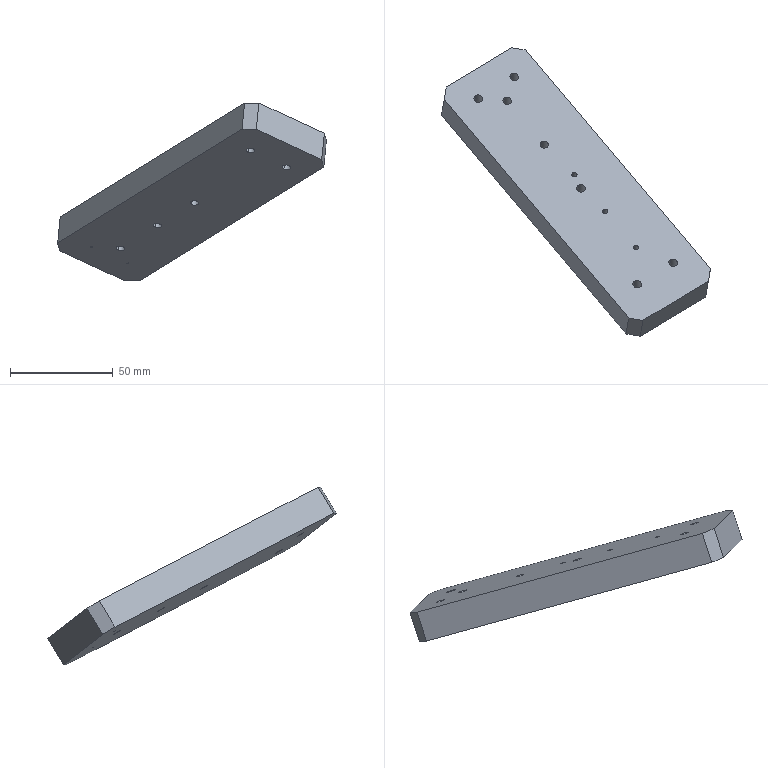Component | SolidWorks | 14AC-24-1-002-1 | 1 solid | 40 faces | box 130.88 x 140.64 x 86.64 mm | volume 117717 mm3 | cylinder 20 | cone 10 | plane 10 | commonest cylinder face diameters 4.2 x12 2.5 x6 4 x2
build123d program:
from build123d import *

# Parameters (mm, degrees)
SKETCH1_W             = 160
SKETCH1_H             = 50
BOSS_EXTRUDE1_DEPTH   = 15
M5_TAPPED_HOLE4_D     = 4.2
CHAMFER1_SIZE         = 5
M5_TAPPED_HOLE2_D     = 4.2
M5_TAPPED_HOLE2_DEPTH = 14
M5_TAPPED_HOLE2_TIP   = 1.262
M5_TAPPED_HOLE3_D     = 4.2
M5_TAPPED_HOLE3_DEPTH = 19
M5_TAPPED_HOLE3_TIP   = 1.262
SKETCH12_R            = 2
CUT_EXTRUDE3_DEPTH    = 163.635
M3_TAPPED_HOLE2_D     = 2.5
M3_TAPPED_HOLE2_DEPTH = 7.5
M3_TAPPED_HOLE2_TIP   = 0.7511


with BuildPart() as part:
    # Sketch1 → Boss-Extrude1 (new body)
    with BuildSketch(Plane.XY):
        with Locations((80, 0)):
            Rectangle(SKETCH1_W, SKETCH1_H)
    extrude(amount=BOSS_EXTRUDE1_DEPTH)

    # M5 Tapped Hole4 (through all)
    with Locations(Plane.XY.offset(15)):
        with Locations((137, 0), (77, 0)):
            Hole(M5_TAPPED_HOLE4_D / 2)

    # Chamfer1
    chamfer1_edges = [part.edges().sort_by_distance(p)[0] for p in [
        (0, 25, 7.5),
        (160, 25, 7.5),
        (160, -25, 7.5),
        (0, -25, 7.5),
    ]]
    chamfer(chamfer1_edges, length=CHAMFER1_SIZE)

    # M5 Tapped Hole2
    with Locations(Plane(origin=(146, -11, 0), x_dir=(-1, 0, 0), z_dir=(0, 0, -1))):
        with Locations((0, 0), (0, 22)):
            Hole(M5_TAPPED_HOLE2_D / 2, depth=M5_TAPPED_HOLE2_DEPTH)
            with Locations((0, 0, -(M5_TAPPED_HOLE2_DEPTH + M5_TAPPED_HOLE2_TIP / 2))):  # 118° drill point
                Cone(0, M5_TAPPED_HOLE2_D / 2, M5_TAPPED_HOLE2_TIP, mode=Mode.SUBTRACT)

    # M5 Tapped Hole3
    with Locations(Plane(origin=(18, -10, 0), x_dir=(-1, 0, 0), z_dir=(0, 0, -1))):
        with Locations((0, 0), (0, 22)):
            Hole(M5_TAPPED_HOLE3_D / 2, depth=M5_TAPPED_HOLE3_DEPTH)
            with Locations((0, 0, -(M5_TAPPED_HOLE3_DEPTH + M5_TAPPED_HOLE3_TIP / 2))):  # 118° drill point
                Cone(0, M5_TAPPED_HOLE3_D / 2, M5_TAPPED_HOLE3_TIP, mode=Mode.SUBTRACT)

    # Sketch12 → Cut-Extrude3 (cut, through all)
    with BuildSketch(Plane.XY.offset(15)):
        with Locations((107, 0)):
            Circle(SKETCH12_R)
    extrude(amount=-CUT_EXTRUDE3_DEPTH, mode=Mode.SUBTRACT)

    # M3 Tapped Hole2
    with Locations(Plane(origin=(0, 0, 0), x_dir=(-1, 0, 0), z_dir=(0, 0, -1))):
        with Locations((-35, 2), (-60, 2), (-85, 2)):
            Hole(M3_TAPPED_HOLE2_D / 2, depth=M3_TAPPED_HOLE2_DEPTH)
            with Locations((0, 0, -(M3_TAPPED_HOLE2_DEPTH + M3_TAPPED_HOLE2_TIP / 2))):  # 118° drill point
                Cone(0, M3_TAPPED_HOLE2_D / 2, M3_TAPPED_HOLE2_TIP, mode=Mode.SUBTRACT)


solid = part.part

# Placed as in the assembly
solid = solid.moved(Location((533.627, -326.914, -38.572), (148.871, -4.92, -126.918)))